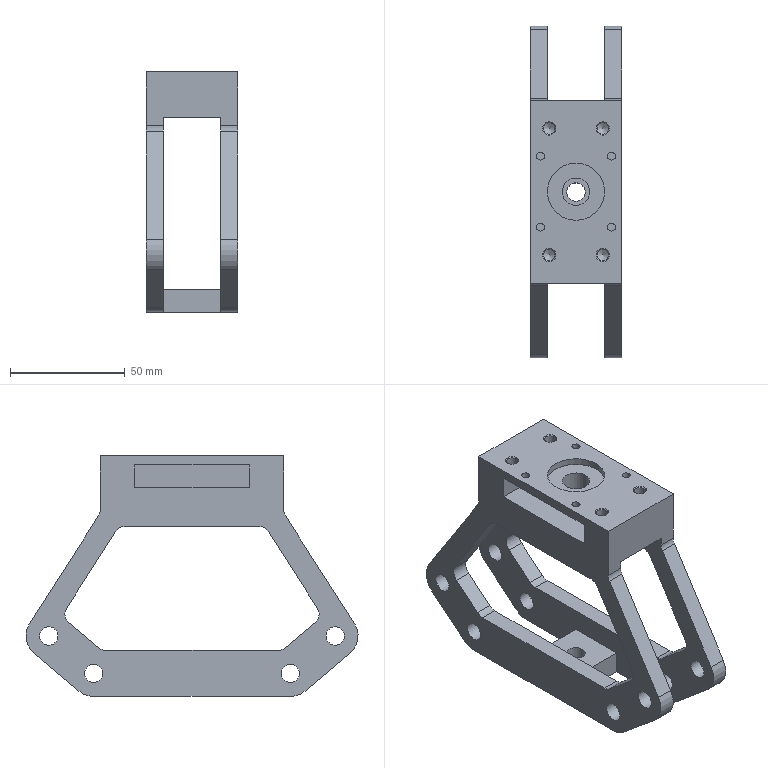Component | NX | BRACKET | 1 solid | 94 faces | volume 125328 mm3 | plane 43 | cylinder 43 | cone 8 | commonest cylinder face diameters 10 x16 8 x9 20 x8 3.5 x4 5 x4 25 x1 12 x1